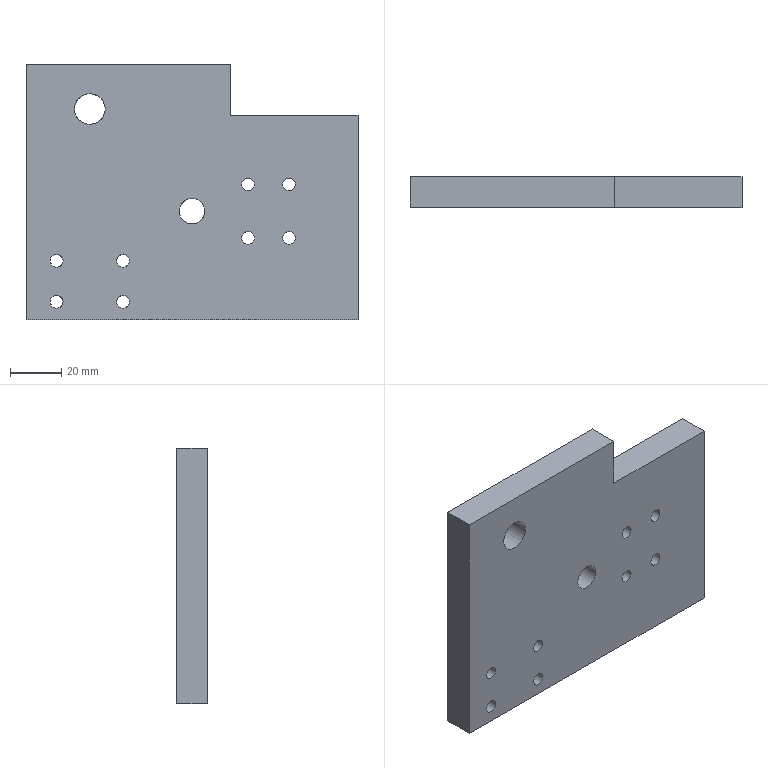Component | NX | VERTICAL_PLATE | 1 solid | 22 faces | volume 139168 mm3 | cylinder 12 | plane 8 | cone 2 | commonest cylinder face diameters 5 x10 12 x1 10 x1